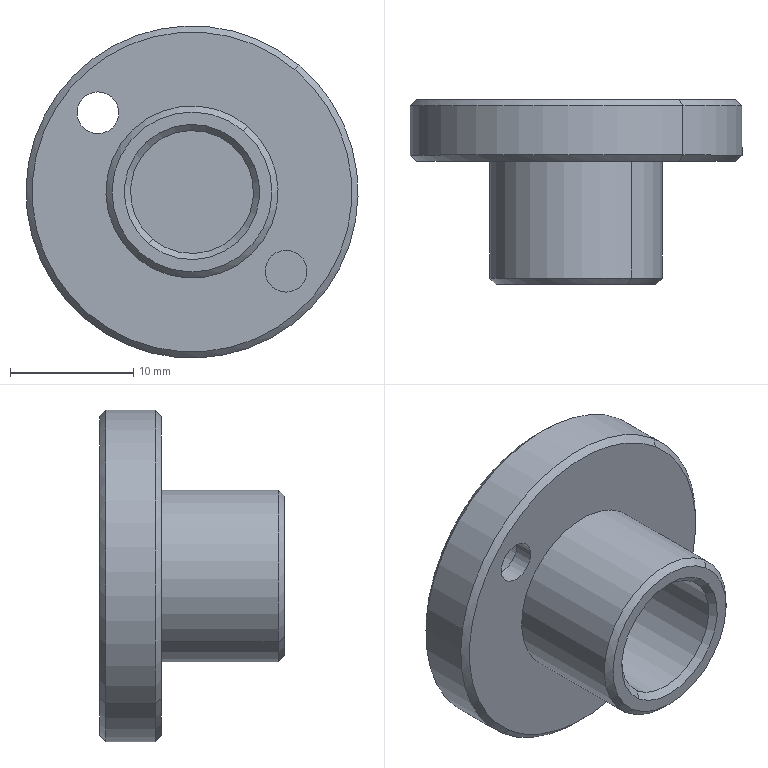Component | SolidWorks | 13LocatingSleeve-1 | 1 solid | 29 faces | box 27 x 15 x 27 mm | volume 2965 mm3 | cylinder 14 | cone 8 | plane 5 | torus 2 | commonest cylinder face diameters 6 x4 3.4 x4 27 x2 10 x2 14 x2 | material 45(Ni)
STEP:
#1=CARTESIAN_POINT('',(-3.318,7.86,-7.582));
#2=VERTEX_POINT('',#1);
#3=CARTESIAN_POINT('',(-2.988,7.86,-7.191));
#4=VERTEX_POINT('',#3);
#5=CARTESIAN_POINT('',(-3.153,7.86,-7.386));
#6=DIRECTION('',(-0.,-1.,-0.));
#7=DIRECTION('',(0.6441,0.,0.765));
#8=AXIS2_PLACEMENT_3D('',#5,#6,#7);
#9=CIRCLE('',#8,0.2559);
#10=EDGE_CURVE('',#2,#4,#9,.T.);
#11=ORIENTED_EDGE('',*,*,#10,.F.);
#12=CARTESIAN_POINT('',(-3.33,7.88,-7.597));
#13=VERTEX_POINT('',#12);
#14=CARTESIAN_POINT('',(-3.33,7.88,-7.597));
#15=DIRECTION('',(-0.4554,0.7071,-0.5409));
#16=VECTOR('',#15,39.37);
#17=LINE('',#14,#16);
#18=EDGE_CURVE('',#2,#13,#17,.T.);
#19=ORIENTED_EDGE('',*,*,#18,.T.);
#20=CARTESIAN_POINT('',(-2.975,7.88,-7.175));
#21=VERTEX_POINT('',#20);
#22=CARTESIAN_POINT('',(-3.153,7.88,-7.386));
#23=DIRECTION('',(0.,1.,0.));
#24=DIRECTION('',(0.6441,0.,0.765));
#25=AXIS2_PLACEMENT_3D('',#22,#23,#24);
#26=CIRCLE('',#25,0.2756);
#27=EDGE_CURVE('',#21,#13,#26,.T.);
#28=ORIENTED_EDGE('',*,*,#27,.F.);
#29=CARTESIAN_POINT('',(-2.975,7.88,-7.175));
#30=DIRECTION('',(0.4554,0.7071,0.5409));
#31=VECTOR('',#30,39.37);
#32=LINE('',#29,#31);
#33=EDGE_CURVE('',#4,#21,#32,.T.);
#34=ORIENTED_EDGE('',*,*,#33,.F.);
#35=EDGE_LOOP('',(#11,#19,#28,#34));
#36=FACE_OUTER_BOUND('',#35,.T.);
#37=CARTESIAN_POINT('',(-3.153,7.88,-7.386));
#38=DIRECTION('',(0.,1.,0.));
#39=DIRECTION('',(0.6441,0.,0.765));
#40=AXIS2_PLACEMENT_3D('',#37,#38,#39);
#41=CONICAL_SURFACE('',#40,0.2756,0.7854);
#42=ADVANCED_FACE('',(#36),#41,.T.);
#43=CARTESIAN_POINT('',(-3.026,7.88,-7.236));
#44=VERTEX_POINT('',#43);
#45=CARTESIAN_POINT('',(-3.28,7.88,-7.537));
#46=VERTEX_POINT('',#45);
#47=CARTESIAN_POINT('',(-3.153,7.88,-7.386));
#48=DIRECTION('',(-0.,-1.,-0.));
#49=DIRECTION('',(0.6441,0.,0.765));
#50=AXIS2_PLACEMENT_3D('',#47,#48,#49);
#51=CIRCLE('',#50,0.1969);
#52=EDGE_CURVE('',#44,#46,#51,.T.);
#53=ORIENTED_EDGE('',*,*,#52,.F.);
#54=CARTESIAN_POINT('',(-3.013,7.86,-7.221));
#55=VERTEX_POINT('',#54);
#56=CARTESIAN_POINT('',(-3.013,7.86,-7.221));
#57=DIRECTION('',(0.4554,-0.7071,0.5409));
#58=VECTOR('',#57,39.37);
#59=LINE('',#56,#58);
#60=EDGE_CURVE('',#44,#55,#59,.T.);
#61=ORIENTED_EDGE('',*,*,#60,.T.);
#62=CARTESIAN_POINT('',(-3.292,7.86,-7.552));
#63=VERTEX_POINT('',#62);
#64=CARTESIAN_POINT('',(-3.153,7.86,-7.386));
#65=DIRECTION('',(0.,1.,0.));
#66=DIRECTION('',(0.6441,0.,0.765));
#67=AXIS2_PLACEMENT_3D('',#64,#65,#66);
#68=CIRCLE('',#67,0.2165);
#69=EDGE_CURVE('',#63,#55,#68,.T.);
#70=ORIENTED_EDGE('',*,*,#69,.F.);
#71=CARTESIAN_POINT('',(-3.292,7.86,-7.552));
#72=DIRECTION('',(-0.4554,-0.7071,-0.5409));
#73=VECTOR('',#72,39.37);
#74=LINE('',#71,#73);
#75=EDGE_CURVE('',#46,#63,#74,.T.);
#76=ORIENTED_EDGE('',*,*,#75,.F.);
#77=EDGE_LOOP('',(#53,#61,#70,#76));
#78=FACE_OUTER_BOUND('',#77,.T.);
#79=CARTESIAN_POINT('',(-3.153,7.86,-7.386));
#80=DIRECTION('',(-0.,-1.,-0.));
#81=DIRECTION('',(-0.6441,0.,-0.765));
#82=AXIS2_PLACEMENT_3D('',#79,#80,#81);
#83=CONICAL_SURFACE('',#82,0.2165,0.7854);
#84=ADVANCED_FACE('',(#78),#83,.F.);
#85=CARTESIAN_POINT('',(-3.482,8.254,-7.778));
#86=VERTEX_POINT('',#85);
#87=CARTESIAN_POINT('',(-2.823,8.254,-6.995));
#88=VERTEX_POINT('',#87);
#89=CARTESIAN_POINT('',(-3.153,8.254,-7.386));
#90=DIRECTION('',(-0.,-1.,-0.));
#91=DIRECTION('',(0.6441,0.,0.765));
#92=AXIS2_PLACEMENT_3D('',#89,#90,#91);
#93=CIRCLE('',#92,0.5118);
#94=EDGE_CURVE('',#86,#88,#93,.T.);
#95=ORIENTED_EDGE('',*,*,#94,.F.);
#96=CARTESIAN_POINT('',(-3.495,8.273,-7.793));
#97=VERTEX_POINT('',#96);
#98=CARTESIAN_POINT('',(-3.495,8.273,-7.793));
#99=DIRECTION('',(-0.4554,0.7071,-0.5409));
#100=VECTOR('',#99,39.37);
#101=LINE('',#98,#100);
#102=EDGE_CURVE('',#86,#97,#101,.T.);
#103=ORIENTED_EDGE('',*,*,#102,.T.);
#104=CARTESIAN_POINT('',(-2.811,8.273,-6.98));
#105=VERTEX_POINT('',#104);
#106=CARTESIAN_POINT('',(-3.153,8.273,-7.386));
#107=DIRECTION('',(0.,1.,0.));
#108=DIRECTION('',(0.6441,0.,0.765));
#109=AXIS2_PLACEMENT_3D('',#106,#107,#108);
#110=CIRCLE('',#109,0.5315);
#111=EDGE_CURVE('',#105,#97,#110,.T.);
#112=ORIENTED_EDGE('',*,*,#111,.F.);
#113=CARTESIAN_POINT('',(-2.811,8.273,-6.98));
#114=DIRECTION('',(0.4554,0.7071,0.5409));
#115=VECTOR('',#114,39.37);
#116=LINE('',#113,#115);
#117=EDGE_CURVE('',#88,#105,#116,.T.);
#118=ORIENTED_EDGE('',*,*,#117,.F.);
#119=EDGE_LOOP('',(#95,#103,#112,#118));
#120=FACE_OUTER_BOUND('',#119,.T.);
#121=CARTESIAN_POINT('',(-3.153,8.273,-7.386));
#122=DIRECTION('',(0.,1.,0.));
#123=DIRECTION('',(0.6441,0.,0.765));
#124=AXIS2_PLACEMENT_3D('',#121,#122,#123);
#125=CONICAL_SURFACE('',#124,0.5315,0.7854);
#126=ADVANCED_FACE('',(#120),#125,.T.);
#127=CARTESIAN_POINT('',(-2.823,8.451,-6.995));
#128=VERTEX_POINT('',#127);
#129=CARTESIAN_POINT('',(-2.761,8.451,-7.716));
#130=VERTEX_POINT('',#129);
#131=CARTESIAN_POINT('',(-3.153,8.451,-7.386));
#132=DIRECTION('',(0.,1.,0.));
#133=DIRECTION('',(0.6441,0.,0.765));
#134=AXIS2_PLACEMENT_3D('',#131,#132,#133);
#135=CIRCLE('',#134,0.5118);
#136=EDGE_CURVE('',#128,#130,#135,.T.);
#137=ORIENTED_EDGE('',*,*,#136,.F.);
#138=CARTESIAN_POINT('',(-2.811,8.431,-6.98));
#139=VERTEX_POINT('',#138);
#140=CARTESIAN_POINT('',(-2.823,8.451,-6.995));
#141=DIRECTION('',(0.4554,-0.7071,0.5409));
#142=VECTOR('',#141,39.37);
#143=LINE('',#140,#142);
#144=EDGE_CURVE('',#128,#139,#143,.T.);
#145=ORIENTED_EDGE('',*,*,#144,.T.);
#146=CARTESIAN_POINT('',(-3.495,8.431,-7.793));
#147=VERTEX_POINT('',#146);
#148=CARTESIAN_POINT('',(-3.153,8.431,-7.386));
#149=DIRECTION('',(-0.,-1.,-0.));
#150=DIRECTION('',(0.6441,0.,0.765));
#151=AXIS2_PLACEMENT_3D('',#148,#149,#150);
#152=CIRCLE('',#151,0.5315);
#153=EDGE_CURVE('',#147,#139,#152,.T.);
#154=ORIENTED_EDGE('',*,*,#153,.F.);
#155=CARTESIAN_POINT('',(-3.482,8.451,-7.778));
#156=VERTEX_POINT('',#155);
#157=CARTESIAN_POINT('',(-3.482,8.451,-7.778));
#158=DIRECTION('',(-0.4554,-0.7071,-0.5409));
#159=VECTOR('',#158,39.37);
#160=LINE('',#157,#159);
#161=EDGE_CURVE('',#156,#147,#160,.T.);
#162=ORIENTED_EDGE('',*,*,#161,.F.);
#163=CARTESIAN_POINT('',(-3.153,8.451,-7.386));
#164=DIRECTION('',(0.,1.,0.));
#165=DIRECTION('',(0.6441,0.,0.765));
#166=AXIS2_PLACEMENT_3D('',#163,#164,#165);
#167=CIRCLE('',#166,0.5118);
#168=EDGE_CURVE('',#130,#156,#167,.T.);
#169=ORIENTED_EDGE('',*,*,#168,.F.);
#170=EDGE_LOOP('',(#137,#145,#154,#162,#169));
#171=FACE_OUTER_BOUND('',#170,.T.);
#172=CARTESIAN_POINT('',(-3.153,8.451,-7.386));
#173=DIRECTION('',(-0.,-1.,-0.));
#174=DIRECTION('',(-0.6441,0.,-0.765));
#175=AXIS2_PLACEMENT_3D('',#172,#173,#174);
#176=CONICAL_SURFACE('',#175,0.5118,0.7854);
#177=ADVANCED_FACE('',(#171),#176,.T.);
#178=CARTESIAN_POINT('',(-3.305,8.451,-7.567));
#179=VERTEX_POINT('',#178);
#180=CARTESIAN_POINT('',(-3.001,8.451,-7.206));
#181=VERTEX_POINT('',#180);
#182=CARTESIAN_POINT('',(-3.153,8.451,-7.386));
#183=DIRECTION('',(-0.,-1.,-0.));
#184=DIRECTION('',(0.6441,0.,0.765));
#185=AXIS2_PLACEMENT_3D('',#182,#183,#184);
#186=CIRCLE('',#185,0.2362);
#187=EDGE_CURVE('',#179,#181,#186,.T.);
#188=ORIENTED_EDGE('',*,*,#187,.F.);
#189=CARTESIAN_POINT('',(-3.28,8.411,-7.537));
#190=VERTEX_POINT('',#189);
#191=CARTESIAN_POINT('',(-3.305,8.411,-7.567));
#192=DIRECTION('',(0.765,0.,-0.6441));
#193=DIRECTION('',(-0.6441,0.,-0.765));
#194=AXIS2_PLACEMENT_3D('',#191,#192,#193);
#195=CIRCLE('',#194,0.03937);
#196=EDGE_CURVE('',#179,#190,#195,.T.);
#197=ORIENTED_EDGE('',*,*,#196,.T.);
#198=CARTESIAN_POINT('',(-3.026,8.411,-7.236));
#199=VERTEX_POINT('',#198);
#200=CARTESIAN_POINT('',(-3.153,8.411,-7.386));
#201=DIRECTION('',(0.,1.,0.));
#202=DIRECTION('',(0.6441,0.,0.765));
#203=AXIS2_PLACEMENT_3D('',#200,#201,#202);
#204=CIRCLE('',#203,0.1969);
#205=EDGE_CURVE('',#199,#190,#204,.T.);
#206=ORIENTED_EDGE('',*,*,#205,.F.);
#207=CARTESIAN_POINT('',(-3.001,8.411,-7.206));
#208=DIRECTION('',(-0.765,-0.,0.6441));
#209=DIRECTION('',(0.6441,0.,0.765));
#210=AXIS2_PLACEMENT_3D('',#207,#208,#209);
#211=CIRCLE('',#210,0.03937);
#212=EDGE_CURVE('',#181,#199,#211,.T.);
#213=ORIENTED_EDGE('',*,*,#212,.F.);
#214=EDGE_LOOP('',(#188,#197,#206,#213));
#215=FACE_OUTER_BOUND('',#214,.T.);
#216=CARTESIAN_POINT('',(-3.153,8.411,-7.386));
#217=DIRECTION('',(0.,1.,0.));
#218=DIRECTION('',(0.6441,-0.,0.765));
#219=AXIS2_PLACEMENT_3D('',#216,#217,#218);
#220=TOROIDAL_SURFACE('',#219,0.2362,0.03937);
#221=ADVANCED_FACE('',(#215),#220,.T.);
#222=CARTESIAN_POINT('',(-2.928,8.317,-7.73));
#223=VERTEX_POINT('',#222);
#224=CARTESIAN_POINT('',(-2.776,8.317,-7.55));
#225=VERTEX_POINT('',#224);
#226=CARTESIAN_POINT('',(-2.852,8.317,-7.64));
#227=DIRECTION('',(0.,1.,0.));
#228=DIRECTION('',(0.6441,0.,0.765));
#229=AXIS2_PLACEMENT_3D('',#226,#227,#228);
#230=CIRCLE('',#229,0.1181);
#231=EDGE_CURVE('',#223,#225,#230,.T.);
#232=ORIENTED_EDGE('',*,*,#231,.F.);
#233=CARTESIAN_POINT('',(-2.928,8.451,-7.73));
#234=VERTEX_POINT('',#233);
#235=CARTESIAN_POINT('',(-2.928,8.451,-7.73));
#236=DIRECTION('',(0.,1.,0.));
#237=VECTOR('',#236,39.37);
#238=LINE('',#235,#237);
#239=EDGE_CURVE('',#223,#234,#238,.T.);
#240=ORIENTED_EDGE('',*,*,#239,.T.);
#241=CARTESIAN_POINT('',(-2.776,8.451,-7.55));
#242=VERTEX_POINT('',#241);
#243=CARTESIAN_POINT('',(-2.852,8.451,-7.64));
#244=DIRECTION('',(0.,1.,0.));
#245=DIRECTION('',(0.6441,0.,0.765));
#246=AXIS2_PLACEMENT_3D('',#243,#244,#245);
#247=CIRCLE('',#246,0.1181);
#248=EDGE_CURVE('',#234,#242,#247,.T.);
#249=ORIENTED_EDGE('',*,*,#248,.T.);
#250=CARTESIAN_POINT('',(-2.776,8.451,-7.55));
#251=DIRECTION('',(0.,1.,0.));
#252=VECTOR('',#251,39.37);
#253=LINE('',#250,#252);
#254=EDGE_CURVE('',#225,#242,#253,.T.);
#255=ORIENTED_EDGE('',*,*,#254,.F.);
#256=EDGE_LOOP('',(#232,#240,#249,#255));
#257=FACE_OUTER_BOUND('',#256,.T.);
#258=CARTESIAN_POINT('',(-2.852,8.451,-7.64));
#259=DIRECTION('',(0.,1.,0.));
#260=DIRECTION('',(0.6441,0.,0.765));
#261=AXIS2_PLACEMENT_3D('',#258,#259,#260);
#262=CYLINDRICAL_SURFACE('',#261,0.1181);
#263=ADVANCED_FACE('',(#257),#262,.F.);
#264=CARTESIAN_POINT('',(-2.895,8.254,-7.691));
#265=VERTEX_POINT('',#264);
#266=CARTESIAN_POINT('',(-2.809,8.254,-7.589));
#267=VERTEX_POINT('',#266);
#268=CARTESIAN_POINT('',(-2.852,8.254,-7.64));
#269=DIRECTION('',(0.,1.,0.));
#270=DIRECTION('',(0.6441,0.,0.765));
#271=AXIS2_PLACEMENT_3D('',#268,#269,#270);
#272=CIRCLE('',#271,0.06693);
#273=EDGE_CURVE('',#265,#267,#272,.T.);
#274=ORIENTED_EDGE('',*,*,#273,.F.);
#275=CARTESIAN_POINT('',(-2.895,8.317,-7.691));
#276=VERTEX_POINT('',#275);
#277=CARTESIAN_POINT('',(-2.895,8.451,-7.691));
#278=DIRECTION('',(0.,1.,0.));
#279=VECTOR('',#278,39.37);
#280=LINE('',#277,#279);
#281=EDGE_CURVE('',#265,#276,#280,.T.);
#282=ORIENTED_EDGE('',*,*,#281,.T.);
#283=CARTESIAN_POINT('',(-2.809,8.317,-7.589));
#284=VERTEX_POINT('',#283);
#285=CARTESIAN_POINT('',(-2.852,8.317,-7.64));
#286=DIRECTION('',(0.,1.,0.));
#287=DIRECTION('',(0.6441,0.,0.765));
#288=AXIS2_PLACEMENT_3D('',#285,#286,#287);
#289=CIRCLE('',#288,0.06693);
#290=EDGE_CURVE('',#276,#284,#289,.T.);
#291=ORIENTED_EDGE('',*,*,#290,.T.);
#292=CARTESIAN_POINT('',(-2.809,8.451,-7.589));
#293=DIRECTION('',(0.,1.,0.));
#294=VECTOR('',#293,39.37);
#295=LINE('',#292,#294);
#296=EDGE_CURVE('',#267,#284,#295,.T.);
#297=ORIENTED_EDGE('',*,*,#296,.F.);
#298=EDGE_LOOP('',(#274,#282,#291,#297));
#299=FACE_OUTER_BOUND('',#298,.T.);
#300=CARTESIAN_POINT('',(-2.852,8.451,-7.64));
#301=DIRECTION('',(0.,1.,0.));
#302=DIRECTION('',(0.6441,0.,0.765));
#303=AXIS2_PLACEMENT_3D('',#300,#301,#302);
#304=CYLINDRICAL_SURFACE('',#303,0.06693);
#305=ADVANCED_FACE('',(#299),#304,.F.);
#306=CARTESIAN_POINT('',(-3.53,8.317,-7.223));
#307=VERTEX_POINT('',#306);
#308=CARTESIAN_POINT('',(-3.378,8.317,-7.042));
#309=VERTEX_POINT('',#308);
#310=CARTESIAN_POINT('',(-3.454,8.317,-7.133));
#311=DIRECTION('',(0.,1.,0.));
#312=DIRECTION('',(0.6441,0.,0.765));
#313=AXIS2_PLACEMENT_3D('',#310,#311,#312);
#314=CIRCLE('',#313,0.1181);
#315=EDGE_CURVE('',#307,#309,#314,.T.);
#316=ORIENTED_EDGE('',*,*,#315,.F.);
#317=CARTESIAN_POINT('',(-3.53,8.451,-7.223));
#318=VERTEX_POINT('',#317);
#319=CARTESIAN_POINT('',(-3.53,8.451,-7.223));
#320=DIRECTION('',(0.,1.,0.));
#321=VECTOR('',#320,39.37);
#322=LINE('',#319,#321);
#323=EDGE_CURVE('',#307,#318,#322,.T.);
#324=ORIENTED_EDGE('',*,*,#323,.T.);
#325=CARTESIAN_POINT('',(-3.544,8.451,-7.057));
#326=VERTEX_POINT('',#325);
#327=CARTESIAN_POINT('',(-3.454,8.451,-7.133));
#328=DIRECTION('',(0.,1.,0.));
#329=DIRECTION('',(0.6441,0.,0.765));
#330=AXIS2_PLACEMENT_3D('',#327,#328,#329);
#331=CIRCLE('',#330,0.1181);
#332=EDGE_CURVE('',#318,#326,#331,.T.);
#333=ORIENTED_EDGE('',*,*,#332,.T.);
#334=CARTESIAN_POINT('',(-3.378,8.451,-7.042));
#335=VERTEX_POINT('',#334);
#336=CARTESIAN_POINT('',(-3.454,8.451,-7.133));
#337=DIRECTION('',(0.,1.,0.));
#338=DIRECTION('',(0.6441,0.,0.765));
#339=AXIS2_PLACEMENT_3D('',#336,#337,#338);
#340=CIRCLE('',#339,0.1181);
#341=EDGE_CURVE('',#326,#335,#340,.T.);
#342=ORIENTED_EDGE('',*,*,#341,.T.);
#343=CARTESIAN_POINT('',(-3.378,8.451,-7.042));
#344=DIRECTION('',(0.,1.,0.));
#345=VECTOR('',#344,39.37);
#346=LINE('',#343,#345);
#347=EDGE_CURVE('',#309,#335,#346,.T.);
#348=ORIENTED_EDGE('',*,*,#347,.F.);
#349=EDGE_LOOP('',(#316,#324,#333,#342,#348));
#350=FACE_OUTER_BOUND('',#349,.T.);
#351=CARTESIAN_POINT('',(-3.454,8.451,-7.133));
#352=DIRECTION('',(0.,1.,0.));
#353=DIRECTION('',(0.6441,0.,0.765));
#354=AXIS2_PLACEMENT_3D('',#351,#352,#353);
#355=CYLINDRICAL_SURFACE('',#354,0.1181);
#356=ADVANCED_FACE('',(#350),#355,.F.);
#357=CARTESIAN_POINT('',(-3.497,8.254,-7.184));
#358=VERTEX_POINT('',#357);
#359=CARTESIAN_POINT('',(-3.411,8.254,-7.082));
#360=VERTEX_POINT('',#359);
#361=CARTESIAN_POINT('',(-3.454,8.254,-7.133));
#362=DIRECTION('',(0.,1.,0.));
#363=DIRECTION('',(0.6441,0.,0.765));
#364=AXIS2_PLACEMENT_3D('',#361,#362,#363);
#365=CIRCLE('',#364,0.06693);
#366=EDGE_CURVE('',#358,#360,#365,.T.);
#367=ORIENTED_EDGE('',*,*,#366,.F.);
#368=CARTESIAN_POINT('',(-3.497,8.317,-7.184));
#369=VERTEX_POINT('',#368);
#370=CARTESIAN_POINT('',(-3.497,8.451,-7.184));
#371=DIRECTION('',(0.,1.,0.));
#372=VECTOR('',#371,39.37);
#373=LINE('',#370,#372);
#374=EDGE_CURVE('',#358,#369,#373,.T.);
#375=ORIENTED_EDGE('',*,*,#374,.T.);
#376=CARTESIAN_POINT('',(-3.411,8.317,-7.082));
#377=VERTEX_POINT('',#376);
#378=CARTESIAN_POINT('',(-3.454,8.317,-7.133));
#379=DIRECTION('',(0.,1.,0.));
#380=DIRECTION('',(0.6441,0.,0.765));
#381=AXIS2_PLACEMENT_3D('',#378,#379,#380);
#382=CIRCLE('',#381,0.06693);
#383=EDGE_CURVE('',#369,#377,#382,.T.);
#384=ORIENTED_EDGE('',*,*,#383,.T.);
#385=CARTESIAN_POINT('',(-3.411,8.451,-7.082));
#386=DIRECTION('',(0.,1.,0.));
#387=VECTOR('',#386,39.37);
#388=LINE('',#385,#387);
#389=EDGE_CURVE('',#360,#377,#388,.T.);
#390=ORIENTED_EDGE('',*,*,#389,.F.);
#391=EDGE_LOOP('',(#367,#375,#384,#390));
#392=FACE_OUTER_BOUND('',#391,.T.);
#393=CARTESIAN_POINT('',(-3.454,8.451,-7.133));
#394=DIRECTION('',(0.,1.,0.));
#395=DIRECTION('',(0.6441,0.,0.765));
#396=AXIS2_PLACEMENT_3D('',#393,#394,#395);
#397=CYLINDRICAL_SURFACE('',#396,0.06693);
#398=ADVANCED_FACE('',(#392),#397,.F.);
#399=ORIENTED_EDGE('',*,*,#111,.T.);
#400=CARTESIAN_POINT('',(-3.495,8.254,-7.793));
#401=DIRECTION('',(0.,1.,0.));
#402=VECTOR('',#401,39.37);
#403=LINE('',#400,#402);
#404=EDGE_CURVE('',#97,#147,#403,.T.);
#405=ORIENTED_EDGE('',*,*,#404,.T.);
#406=ORIENTED_EDGE('',*,*,#153,.T.);
#407=CARTESIAN_POINT('',(-2.811,8.254,-6.98));
#408=DIRECTION('',(0.,1.,0.));
#409=VECTOR('',#408,39.37);
#410=LINE('',#407,#409);
#411=EDGE_CURVE('',#105,#139,#410,.T.);
#412=ORIENTED_EDGE('',*,*,#411,.F.);
#413=EDGE_LOOP('',(#399,#405,#406,#412));
#414=FACE_OUTER_BOUND('',#413,.T.);
#415=CARTESIAN_POINT('',(-3.153,8.254,-7.386));
#416=DIRECTION('',(0.,1.,0.));
#417=DIRECTION('',(0.6441,0.,0.765));
#418=AXIS2_PLACEMENT_3D('',#415,#416,#417);
#419=CYLINDRICAL_SURFACE('',#418,0.5315);
#420=ADVANCED_FACE('',(#414),#419,.T.);
#421=CARTESIAN_POINT('',(-3.153,8.411,-7.386));
#422=DIRECTION('',(0.,1.,0.));
#423=DIRECTION('',(0.6441,0.,0.765));
#424=AXIS2_PLACEMENT_3D('',#421,#422,#423);
#425=CIRCLE('',#424,0.1969);
#426=EDGE_CURVE('',#190,#199,#425,.T.);
#427=ORIENTED_EDGE('',*,*,#426,.T.);
#428=CARTESIAN_POINT('',(-3.026,8.451,-7.236));
#429=DIRECTION('',(-0.,-1.,-0.));
#430=VECTOR('',#429,39.37);
#431=LINE('',#428,#430);
#432=EDGE_CURVE('',#199,#44,#431,.T.);
#433=ORIENTED_EDGE('',*,*,#432,.T.);
#434=ORIENTED_EDGE('',*,*,#52,.T.);
#435=CARTESIAN_POINT('',(-3.28,8.451,-7.537));
#436=DIRECTION('',(-0.,-1.,-0.));
#437=VECTOR('',#436,39.37);
#438=LINE('',#435,#437);
#439=EDGE_CURVE('',#190,#46,#438,.T.);
#440=ORIENTED_EDGE('',*,*,#439,.F.);
#441=EDGE_LOOP('',(#427,#433,#434,#440));
#442=FACE_OUTER_BOUND('',#441,.T.);
#443=CARTESIAN_POINT('',(-3.153,8.451,-7.386));
#444=DIRECTION('',(-0.,-1.,-0.));
#445=DIRECTION('',(-0.6441,0.,-0.765));
#446=AXIS2_PLACEMENT_3D('',#443,#444,#445);
#447=CYLINDRICAL_SURFACE('',#446,0.1969);
#448=ADVANCED_FACE('',(#442),#447,.F.);
#449=CARTESIAN_POINT('',(-2.975,8.254,-7.175));
#450=VERTEX_POINT('',#449);
#451=CARTESIAN_POINT('',(-3.33,8.254,-7.597));
#452=VERTEX_POINT('',#451);
#453=CARTESIAN_POINT('',(-3.153,8.254,-7.386));
#454=DIRECTION('',(0.,1.,0.));
#455=DIRECTION('',(0.6441,0.,0.765));
#456=AXIS2_PLACEMENT_3D('',#453,#454,#455);
#457=CIRCLE('',#456,0.2756);
#458=EDGE_CURVE('',#450,#452,#457,.T.);
#459=ORIENTED_EDGE('',*,*,#458,.F.);
#460=CARTESIAN_POINT('',(-2.975,8.451,-7.175));
#461=DIRECTION('',(-0.,-1.,-0.));
#462=VECTOR('',#461,39.37);
#463=LINE('',#460,#462);
#464=EDGE_CURVE('',#450,#21,#463,.T.);
#465=ORIENTED_EDGE('',*,*,#464,.T.);
#466=ORIENTED_EDGE('',*,*,#27,.T.);
#467=CARTESIAN_POINT('',(-3.33,8.451,-7.597));
#468=DIRECTION('',(-0.,-1.,-0.));
#469=VECTOR('',#468,39.37);
#470=LINE('',#467,#469);
#471=EDGE_CURVE('',#452,#13,#470,.T.);
#472=ORIENTED_EDGE('',*,*,#471,.F.);
#473=EDGE_LOOP('',(#459,#465,#466,#472));
#474=FACE_OUTER_BOUND('',#473,.T.);
#475=CARTESIAN_POINT('',(-3.153,8.451,-7.386));
#476=DIRECTION('',(-0.,-1.,-0.));
#477=DIRECTION('',(-0.6441,0.,-0.765));
#478=AXIS2_PLACEMENT_3D('',#475,#476,#477);
#479=CYLINDRICAL_SURFACE('',#478,0.2756);
#480=ADVANCED_FACE('',(#474),#479,.T.);
#481=ORIENTED_EDGE('',*,*,#464,.F.);
#482=CARTESIAN_POINT('',(-3.153,8.254,-7.386));
#483=DIRECTION('',(0.,1.,0.));
#484=DIRECTION('',(0.6441,0.,0.765));
#485=AXIS2_PLACEMENT_3D('',#482,#483,#484);
#486=CIRCLE('',#485,0.2756);
#487=EDGE_CURVE('',#452,#450,#486,.T.);
#488=ORIENTED_EDGE('',*,*,#487,.F.);
#489=ORIENTED_EDGE('',*,*,#471,.T.);
#490=CARTESIAN_POINT('',(-3.153,7.88,-7.386));
#491=DIRECTION('',(0.,1.,0.));
#492=DIRECTION('',(0.6441,0.,0.765));
#493=AXIS2_PLACEMENT_3D('',#490,#491,#492);
#494=CIRCLE('',#493,0.2756);
#495=EDGE_CURVE('',#13,#21,#494,.T.);
#496=ORIENTED_EDGE('',*,*,#495,.T.);
#497=EDGE_LOOP('',(#481,#488,#489,#496));
#498=FACE_OUTER_BOUND('',#497,.T.);
#499=CARTESIAN_POINT('',(-3.153,8.451,-7.386));
#500=DIRECTION('',(-0.,-1.,-0.));
#501=DIRECTION('',(-0.6441,0.,-0.765));
#502=AXIS2_PLACEMENT_3D('',#499,#500,#501);
#503=CYLINDRICAL_SURFACE('',#502,0.2756);
#504=ADVANCED_FACE('',(#498),#503,.T.);
#505=CARTESIAN_POINT('',(-3.153,8.451,-7.386));
#506=DIRECTION('',(-0.,-1.,-0.));
#507=DIRECTION('',(0.6441,0.,0.765));
#508=AXIS2_PLACEMENT_3D('',#505,#506,#507);
#509=CIRCLE('',#508,0.2362);
#510=EDGE_CURVE('',#181,#179,#509,.T.);
#511=ORIENTED_EDGE('',*,*,#510,.T.);
#512=ORIENTED_EDGE('',*,*,#187,.T.);
#513=EDGE_LOOP('',(#511,#512));
#514=FACE_BOUND('',#513,.T.);
#515=CARTESIAN_POINT('',(-2.852,8.451,-7.64));
#516=DIRECTION('',(0.,1.,0.));
#517=DIRECTION('',(0.6441,0.,0.765));
#518=AXIS2_PLACEMENT_3D('',#515,#516,#517);
#519=CIRCLE('',#518,0.1181);
#520=EDGE_CURVE('',#130,#234,#519,.T.);
#521=ORIENTED_EDGE('',*,*,#520,.F.);
#522=ORIENTED_EDGE('',*,*,#168,.T.);
#523=CARTESIAN_POINT('',(-3.153,8.451,-7.386));
#524=DIRECTION('',(0.,1.,0.));
#525=DIRECTION('',(0.6441,0.,0.765));
#526=AXIS2_PLACEMENT_3D('',#523,#524,#525);
#527=CIRCLE('',#526,0.5118);
#528=EDGE_CURVE('',#156,#326,#527,.T.);
#529=ORIENTED_EDGE('',*,*,#528,.T.);
#530=ORIENTED_EDGE('',*,*,#332,.F.);
#531=CARTESIAN_POINT('',(-3.454,8.451,-7.133));
#532=DIRECTION('',(0.,1.,0.));
#533=DIRECTION('',(0.6441,0.,0.765));
#534=AXIS2_PLACEMENT_3D('',#531,#532,#533);
#535=CIRCLE('',#534,0.1181);
#536=EDGE_CURVE('',#335,#318,#535,.T.);
#537=ORIENTED_EDGE('',*,*,#536,.F.);
#538=ORIENTED_EDGE('',*,*,#341,.F.);
#539=CARTESIAN_POINT('',(-3.153,8.451,-7.386));
#540=DIRECTION('',(0.,1.,0.));
#541=DIRECTION('',(0.6441,0.,0.765));
#542=AXIS2_PLACEMENT_3D('',#539,#540,#541);
#543=CIRCLE('',#542,0.5118);
#544=EDGE_CURVE('',#326,#128,#543,.T.);
#545=ORIENTED_EDGE('',*,*,#544,.T.);
#546=ORIENTED_EDGE('',*,*,#136,.T.);
#547=CARTESIAN_POINT('',(-2.852,8.451,-7.64));
#548=DIRECTION('',(0.,1.,0.));
#549=DIRECTION('',(0.6441,0.,0.765));
#550=AXIS2_PLACEMENT_3D('',#547,#548,#549);
#551=CIRCLE('',#550,0.1181);
#552=EDGE_CURVE('',#242,#130,#551,.T.);
#553=ORIENTED_EDGE('',*,*,#552,.F.);
#554=ORIENTED_EDGE('',*,*,#248,.F.);
#555=EDGE_LOOP('',(#521,#522,#529,#530,#537,#538,#545,#546,#553,#554));
#556=FACE_OUTER_BOUND('',#555,.T.);
#557=CARTESIAN_POINT('',(-3.153,8.451,-7.386));
#558=DIRECTION('',(0.,1.,0.));
#559=DIRECTION('',(0.6441,-0.,0.765));
#560=AXIS2_PLACEMENT_3D('',#557,#558,#559);
#561=PLANE('',#560);
#562=ADVANCED_FACE('',(#514,#556),#561,.T.);
#563=ORIENTED_EDGE('',*,*,#69,.T.);
#564=CARTESIAN_POINT('',(-3.153,7.86,-7.386));
#565=DIRECTION('',(0.,1.,0.));
#566=DIRECTION('',(0.6441,0.,0.765));
#567=AXIS2_PLACEMENT_3D('',#564,#565,#566);
#568=CIRCLE('',#567,0.2165);
#569=EDGE_CURVE('',#55,#63,#568,.T.);
#570=ORIENTED_EDGE('',*,*,#569,.T.);
#571=EDGE_LOOP('',(#563,#570));
#572=FACE_BOUND('',#571,.T.);
#573=CARTESIAN_POINT('',(-3.153,7.86,-7.386));
#574=DIRECTION('',(-0.,-1.,-0.));
#575=DIRECTION('',(0.6441,0.,0.765));
#576=AXIS2_PLACEMENT_3D('',#573,#574,#575);
#577=CIRCLE('',#576,0.2559);
#578=EDGE_CURVE('',#4,#2,#577,.T.);
#579=ORIENTED_EDGE('',*,*,#578,.T.);
#580=ORIENTED_EDGE('',*,*,#10,.T.);
#581=EDGE_LOOP('',(#579,#580));
#582=FACE_OUTER_BOUND('',#581,.T.);
#583=CARTESIAN_POINT('',(-3.153,7.86,-7.386));
#584=DIRECTION('',(0.,1.,0.));
#585=DIRECTION('',(0.6441,-0.,0.765));
#586=AXIS2_PLACEMENT_3D('',#583,#584,#585);
#587=PLANE('',#586);
#588=ADVANCED_FACE('',(#572,#582),#587,.F.);
#589=ORIENTED_EDGE('',*,*,#432,.F.);
#590=ORIENTED_EDGE('',*,*,#205,.T.);
#591=ORIENTED_EDGE('',*,*,#439,.T.);
#592=CARTESIAN_POINT('',(-3.153,7.88,-7.386));
#593=DIRECTION('',(-0.,-1.,-0.));
#594=DIRECTION('',(0.6441,0.,0.765));
#595=AXIS2_PLACEMENT_3D('',#592,#593,#594);
#596=CIRCLE('',#595,0.1969);
#597=EDGE_CURVE('',#46,#44,#596,.T.);
#598=ORIENTED_EDGE('',*,*,#597,.T.);
#599=EDGE_LOOP('',(#589,#590,#591,#598));
#600=FACE_OUTER_BOUND('',#599,.T.);
#601=CARTESIAN_POINT('',(-3.153,8.451,-7.386));
#602=DIRECTION('',(-0.,-1.,-0.));
#603=DIRECTION('',(-0.6441,0.,-0.765));
#604=AXIS2_PLACEMENT_3D('',#601,#602,#603);
#605=CYLINDRICAL_SURFACE('',#604,0.1969);
#606=ADVANCED_FACE('',(#600),#605,.F.);
#607=ORIENTED_EDGE('',*,*,#404,.F.);
#608=CARTESIAN_POINT('',(-3.153,8.273,-7.386));
#609=DIRECTION('',(0.,1.,0.));
#610=DIRECTION('',(0.6441,0.,0.765));
#611=AXIS2_PLACEMENT_3D('',#608,#609,#610);
#612=CIRCLE('',#611,0.5315);
#613=EDGE_CURVE('',#97,#105,#612,.T.);
#614=ORIENTED_EDGE('',*,*,#613,.T.);
#615=ORIENTED_EDGE('',*,*,#411,.T.);
#616=CARTESIAN_POINT('',(-3.153,8.431,-7.386));
#617=DIRECTION('',(-0.,-1.,-0.));
#618=DIRECTION('',(0.6441,0.,0.765));
#619=AXIS2_PLACEMENT_3D('',#616,#617,#618);
#620=CIRCLE('',#619,0.5315);
#621=EDGE_CURVE('',#139,#147,#620,.T.);
#622=ORIENTED_EDGE('',*,*,#621,.T.);
#623=EDGE_LOOP('',(#607,#614,#615,#622));
#624=FACE_OUTER_BOUND('',#623,.T.);
#625=CARTESIAN_POINT('',(-3.153,8.254,-7.386));
#626=DIRECTION('',(0.,1.,0.));
#627=DIRECTION('',(0.6441,0.,0.765));
#628=AXIS2_PLACEMENT_3D('',#625,#626,#627);
#629=CYLINDRICAL_SURFACE('',#628,0.5315);
#630=ADVANCED_FACE('',(#624),#629,.T.);
#631=CARTESIAN_POINT('',(-3.153,8.254,-7.386));
#632=DIRECTION('',(-0.,-1.,-0.));
#633=DIRECTION('',(0.6441,0.,0.765));
#634=AXIS2_PLACEMENT_3D('',#631,#632,#633);
#635=CIRCLE('',#634,0.5118);
#636=EDGE_CURVE('',#88,#86,#635,.T.);
#637=ORIENTED_EDGE('',*,*,#636,.T.);
#638=ORIENTED_EDGE('',*,*,#94,.T.);
#639=EDGE_LOOP('',(#637,#638));
#640=FACE_OUTER_BOUND('',#639,.T.);
#641=CARTESIAN_POINT('',(-2.852,8.254,-7.64));
#642=DIRECTION('',(0.,1.,0.));
#643=DIRECTION('',(0.6441,0.,0.765));
#644=AXIS2_PLACEMENT_3D('',#641,#642,#643);
#645=CIRCLE('',#644,0.06693);
#646=EDGE_CURVE('',#267,#265,#645,.T.);
#647=ORIENTED_EDGE('',*,*,#646,.T.);
#648=ORIENTED_EDGE('',*,*,#273,.T.);
#649=EDGE_LOOP('',(#647,#648));
#650=FACE_BOUND('',#649,.T.);
#651=CARTESIAN_POINT('',(-3.454,8.254,-7.133));
#652=DIRECTION('',(0.,1.,0.));
#653=DIRECTION('',(0.6441,0.,0.765));
#654=AXIS2_PLACEMENT_3D('',#651,#652,#653);
#655=CIRCLE('',#654,0.06693);
#656=EDGE_CURVE('',#360,#358,#655,.T.);
#657=ORIENTED_EDGE('',*,*,#656,.T.);
#658=ORIENTED_EDGE('',*,*,#366,.T.);
#659=EDGE_LOOP('',(#657,#658));
#660=FACE_BOUND('',#659,.T.);
#661=ORIENTED_EDGE('',*,*,#487,.T.);
#662=ORIENTED_EDGE('',*,*,#458,.T.);
#663=EDGE_LOOP('',(#661,#662));
#664=FACE_BOUND('',#663,.T.);
#665=CARTESIAN_POINT('',(-3.153,8.254,-7.386));
#666=DIRECTION('',(0.,1.,0.));
#667=DIRECTION('',(0.6441,-0.,0.765));
#668=AXIS2_PLACEMENT_3D('',#665,#666,#667);
#669=PLANE('',#668);
#670=ADVANCED_FACE('',(#640,#650,#660,#664),#669,.F.);
#671=ORIENTED_EDGE('',*,*,#374,.F.);
#672=ORIENTED_EDGE('',*,*,#656,.F.);
#673=ORIENTED_EDGE('',*,*,#389,.T.);
#674=CARTESIAN_POINT('',(-3.454,8.317,-7.133));
#675=DIRECTION('',(0.,1.,0.));
#676=DIRECTION('',(0.6441,0.,0.765));
#677=AXIS2_PLACEMENT_3D('',#674,#675,#676);
#678=CIRCLE('',#677,0.06693);
#679=EDGE_CURVE('',#377,#369,#678,.T.);
#680=ORIENTED_EDGE('',*,*,#679,.T.);
#681=EDGE_LOOP('',(#671,#672,#673,#680));
#682=FACE_OUTER_BOUND('',#681,.T.);
#683=CARTESIAN_POINT('',(-3.454,8.451,-7.133));
#684=DIRECTION('',(0.,1.,0.));
#685=DIRECTION('',(0.6441,0.,0.765));
#686=AXIS2_PLACEMENT_3D('',#683,#684,#685);
#687=CYLINDRICAL_SURFACE('',#686,0.06693);
#688=ADVANCED_FACE('',(#682),#687,.F.);
#689=ORIENTED_EDGE('',*,*,#679,.F.);
#690=ORIENTED_EDGE('',*,*,#383,.F.);
#691=EDGE_LOOP('',(#689,#690));
#692=FACE_BOUND('',#691,.T.);
#693=CARTESIAN_POINT('',(-3.454,8.317,-7.133));
#694=DIRECTION('',(0.,1.,0.));
#695=DIRECTION('',(0.6441,0.,0.765));
#696=AXIS2_PLACEMENT_3D('',#693,#694,#695);
#697=CIRCLE('',#696,0.1181);
#698=EDGE_CURVE('',#309,#307,#697,.T.);
#699=ORIENTED_EDGE('',*,*,#698,.T.);
#700=ORIENTED_EDGE('',*,*,#315,.T.);
#701=EDGE_LOOP('',(#699,#700));
#702=FACE_OUTER_BOUND('',#701,.T.);
#703=CARTESIAN_POINT('',(-3.411,8.317,-7.082));
#704=DIRECTION('',(-0.,-1.,-0.));
#705=DIRECTION('',(-0.6441,0.,-0.765));
#706=AXIS2_PLACEMENT_3D('',#703,#704,#705);
#707=PLANE('',#706);
#708=ADVANCED_FACE('',(#692,#702),#707,.F.);
#709=ORIENTED_EDGE('',*,*,#323,.F.);
#710=ORIENTED_EDGE('',*,*,#698,.F.);
#711=ORIENTED_EDGE('',*,*,#347,.T.);
#712=ORIENTED_EDGE('',*,*,#536,.T.);
#713=EDGE_LOOP('',(#709,#710,#711,#712));
#714=FACE_OUTER_BOUND('',#713,.T.);
#715=CARTESIAN_POINT('',(-3.454,8.451,-7.133));
#716=DIRECTION('',(0.,1.,0.));
#717=DIRECTION('',(0.6441,0.,0.765));
#718=AXIS2_PLACEMENT_3D('',#715,#716,#717);
#719=CYLINDRICAL_SURFACE('',#718,0.1181);
#720=ADVANCED_FACE('',(#714),#719,.F.);
#721=ORIENTED_EDGE('',*,*,#281,.F.);
#722=ORIENTED_EDGE('',*,*,#646,.F.);
#723=ORIENTED_EDGE('',*,*,#296,.T.);
#724=CARTESIAN_POINT('',(-2.852,8.317,-7.64));
#725=DIRECTION('',(0.,1.,0.));
#726=DIRECTION('',(0.6441,0.,0.765));
#727=AXIS2_PLACEMENT_3D('',#724,#725,#726);
#728=CIRCLE('',#727,0.06693);
#729=EDGE_CURVE('',#284,#276,#728,.T.);
#730=ORIENTED_EDGE('',*,*,#729,.T.);
#731=EDGE_LOOP('',(#721,#722,#723,#730));
#732=FACE_OUTER_BOUND('',#731,.T.);
#733=CARTESIAN_POINT('',(-2.852,8.451,-7.64));
#734=DIRECTION('',(0.,1.,0.));
#735=DIRECTION('',(0.6441,0.,0.765));
#736=AXIS2_PLACEMENT_3D('',#733,#734,#735);
#737=CYLINDRICAL_SURFACE('',#736,0.06693);
#738=ADVANCED_FACE('',(#732),#737,.F.);
#739=ORIENTED_EDGE('',*,*,#729,.F.);
#740=ORIENTED_EDGE('',*,*,#290,.F.);
#741=EDGE_LOOP('',(#739,#740));
#742=FACE_BOUND('',#741,.T.);
#743=CARTESIAN_POINT('',(-2.852,8.317,-7.64));
#744=DIRECTION('',(0.,1.,0.));
#745=DIRECTION('',(0.6441,0.,0.765));
#746=AXIS2_PLACEMENT_3D('',#743,#744,#745);
#747=CIRCLE('',#746,0.1181);
#748=EDGE_CURVE('',#225,#223,#747,.T.);
#749=ORIENTED_EDGE('',*,*,#748,.T.);
#750=ORIENTED_EDGE('',*,*,#231,.T.);
#751=EDGE_LOOP('',(#749,#750));
#752=FACE_OUTER_BOUND('',#751,.T.);
#753=CARTESIAN_POINT('',(-2.809,8.317,-7.589));
#754=DIRECTION('',(-0.,-1.,-0.));
#755=DIRECTION('',(-0.6441,0.,-0.765));
#756=AXIS2_PLACEMENT_3D('',#753,#754,#755);
#757=PLANE('',#756);
#758=ADVANCED_FACE('',(#742,#752),#757,.F.);
#759=ORIENTED_EDGE('',*,*,#239,.F.);
#760=ORIENTED_EDGE('',*,*,#748,.F.);
#761=ORIENTED_EDGE('',*,*,#254,.T.);
#762=ORIENTED_EDGE('',*,*,#552,.T.);
#763=ORIENTED_EDGE('',*,*,#520,.T.);
#764=EDGE_LOOP('',(#759,#760,#761,#762,#763));
#765=FACE_OUTER_BOUND('',#764,.T.);
#766=CARTESIAN_POINT('',(-2.852,8.451,-7.64));
#767=DIRECTION('',(0.,1.,0.));
#768=DIRECTION('',(0.6441,0.,0.765));
#769=AXIS2_PLACEMENT_3D('',#766,#767,#768);
#770=CYLINDRICAL_SURFACE('',#769,0.1181);
#771=ADVANCED_FACE('',(#765),#770,.F.);
#772=ORIENTED_EDGE('',*,*,#196,.F.);
#773=ORIENTED_EDGE('',*,*,#510,.F.);
#774=ORIENTED_EDGE('',*,*,#212,.T.);
#775=ORIENTED_EDGE('',*,*,#426,.F.);
#776=EDGE_LOOP('',(#772,#773,#774,#775));
#777=FACE_OUTER_BOUND('',#776,.T.);
#778=CARTESIAN_POINT('',(-3.153,8.411,-7.386));
#779=DIRECTION('',(0.,1.,0.));
#780=DIRECTION('',(0.6441,-0.,0.765));
#781=AXIS2_PLACEMENT_3D('',#778,#779,#780);
#782=TOROIDAL_SURFACE('',#781,0.2362,0.03937);
#783=ADVANCED_FACE('',(#777),#782,.T.);
#784=ORIENTED_EDGE('',*,*,#144,.F.);
#785=ORIENTED_EDGE('',*,*,#544,.F.);
#786=ORIENTED_EDGE('',*,*,#528,.F.);
#787=ORIENTED_EDGE('',*,*,#161,.T.);
#788=ORIENTED_EDGE('',*,*,#621,.F.);
#789=EDGE_LOOP('',(#784,#785,#786,#787,#788));
#790=FACE_OUTER_BOUND('',#789,.T.);
#791=CARTESIAN_POINT('',(-3.153,8.451,-7.386));
#792=DIRECTION('',(-0.,-1.,-0.));
#793=DIRECTION('',(-0.6441,0.,-0.765));
#794=AXIS2_PLACEMENT_3D('',#791,#792,#793);
#795=CONICAL_SURFACE('',#794,0.5118,0.7854);
#796=ADVANCED_FACE('',(#790),#795,.T.);
#797=ORIENTED_EDGE('',*,*,#102,.F.);
#798=ORIENTED_EDGE('',*,*,#636,.F.);
#799=ORIENTED_EDGE('',*,*,#117,.T.);
#800=ORIENTED_EDGE('',*,*,#613,.F.);
#801=EDGE_LOOP('',(#797,#798,#799,#800));
#802=FACE_OUTER_BOUND('',#801,.T.);
#803=CARTESIAN_POINT('',(-3.153,8.273,-7.386));
#804=DIRECTION('',(0.,1.,0.));
#805=DIRECTION('',(0.6441,0.,0.765));
#806=AXIS2_PLACEMENT_3D('',#803,#804,#805);
#807=CONICAL_SURFACE('',#806,0.5315,0.7854);
#808=ADVANCED_FACE('',(#802),#807,.T.);
#809=ORIENTED_EDGE('',*,*,#60,.F.);
#810=ORIENTED_EDGE('',*,*,#597,.F.);
#811=ORIENTED_EDGE('',*,*,#75,.T.);
#812=ORIENTED_EDGE('',*,*,#569,.F.);
#813=EDGE_LOOP('',(#809,#810,#811,#812));
#814=FACE_OUTER_BOUND('',#813,.T.);
#815=CARTESIAN_POINT('',(-3.153,7.86,-7.386));
#816=DIRECTION('',(-0.,-1.,-0.));
#817=DIRECTION('',(-0.6441,0.,-0.765));
#818=AXIS2_PLACEMENT_3D('',#815,#816,#817);
#819=CONICAL_SURFACE('',#818,0.2165,0.7854);
#820=ADVANCED_FACE('',(#814),#819,.F.);
#821=ORIENTED_EDGE('',*,*,#18,.F.);
#822=ORIENTED_EDGE('',*,*,#578,.F.);
#823=ORIENTED_EDGE('',*,*,#33,.T.);
#824=ORIENTED_EDGE('',*,*,#495,.F.);
#825=EDGE_LOOP('',(#821,#822,#823,#824));
#826=FACE_OUTER_BOUND('',#825,.T.);
#827=CARTESIAN_POINT('',(-3.153,7.88,-7.386));
#828=DIRECTION('',(0.,1.,0.));
#829=DIRECTION('',(0.6441,0.,0.765));
#830=AXIS2_PLACEMENT_3D('',#827,#828,#829);
#831=CONICAL_SURFACE('',#830,0.2756,0.7854);
#832=ADVANCED_FACE('',(#826),#831,.T.);
#833=CLOSED_SHELL('',(#42,#84,#126,#177,#221,#263,#305,#356,#398,#420,#448,#480,#504,#562,#588,#606,#630,#670,#688,#708,#720,#738,#758,#771,#783,#796,#808,#820,#832));
#834=MANIFOLD_SOLID_BREP('',#833);
#835=CARTESIAN_POINT('',(0.,0.,0.));
#836=DIRECTION('',(0.,0.,1.));
#837=DIRECTION('',(1.,0.,0.));
#838=AXIS2_PLACEMENT_3D('',#835,#836,#837);
#839=(LENGTH_UNIT()NAMED_UNIT(*)SI_UNIT($,.METRE.));
#840=LENGTH_MEASURE_WITH_UNIT(LENGTH_MEASURE(0.0254),#839);
#841=DIMENSIONAL_EXPONENTS(1.,0.,0.,0.,0.,0.,0.);
#842=(CONVERSION_BASED_UNIT('',#840)LENGTH_UNIT()NAMED_UNIT(#841));
#843=UNCERTAINTY_MEASURE_WITH_UNIT(LENGTH_MEASURE(0.00001),#842,'','');
#844=(NAMED_UNIT(*)PLANE_ANGLE_UNIT()SI_UNIT($,.RADIAN.));
#845=(NAMED_UNIT(*)SI_UNIT($,.STERADIAN.)SOLID_ANGLE_UNIT());
#846=(GEOMETRIC_REPRESENTATION_CONTEXT(3)GLOBAL_UNCERTAINTY_ASSIGNED_CONTEXT((#843))GLOBAL_UNIT_ASSIGNED_CONTEXT((#842,#844,#845))REPRESENTATION_CONTEXT('',''));
#847=ADVANCED_BREP_SHAPE_REPRESENTATION('',(#834,#838),#846);
#848=COLOUR_RGB('',0.7922,0.8196,0.9333);
#849=FILL_AREA_STYLE_COLOUR('',#848);
#850=FILL_AREA_STYLE('',(#849));
#851=SURFACE_STYLE_FILL_AREA(#850);
#852=SURFACE_SIDE_STYLE('',(#851));
#853=SURFACE_STYLE_USAGE(.BOTH.,#852);
#854=PRESENTATION_STYLE_ASSIGNMENT((#853));
#855=STYLED_ITEM('',(#854),#834);
#856=(LENGTH_UNIT()NAMED_UNIT(*)SI_UNIT($,.METRE.));
#857=LENGTH_MEASURE_WITH_UNIT(LENGTH_MEASURE(0.0254),#856);
#858=DIMENSIONAL_EXPONENTS(1.,0.,0.,0.,0.,0.,0.);
#859=(CONVERSION_BASED_UNIT('',#857)LENGTH_UNIT()NAMED_UNIT(#858));
#860=UNCERTAINTY_MEASURE_WITH_UNIT(LENGTH_MEASURE(0.00001),#859,'','');
#861=(NAMED_UNIT(*)PLANE_ANGLE_UNIT()SI_UNIT($,.RADIAN.));
#862=(NAMED_UNIT(*)SI_UNIT($,.STERADIAN.)SOLID_ANGLE_UNIT());
#863=(GEOMETRIC_REPRESENTATION_CONTEXT(3)GLOBAL_UNCERTAINTY_ASSIGNED_CONTEXT((#860))GLOBAL_UNIT_ASSIGNED_CONTEXT((#859,#861,#862))REPRESENTATION_CONTEXT('',''));
#864=MECHANICAL_DESIGN_GEOMETRIC_PRESENTATION_REPRESENTATION('',(#855),#863);
#865=PRESENTATION_LAYER_ASSIGNMENT('','',(#855));